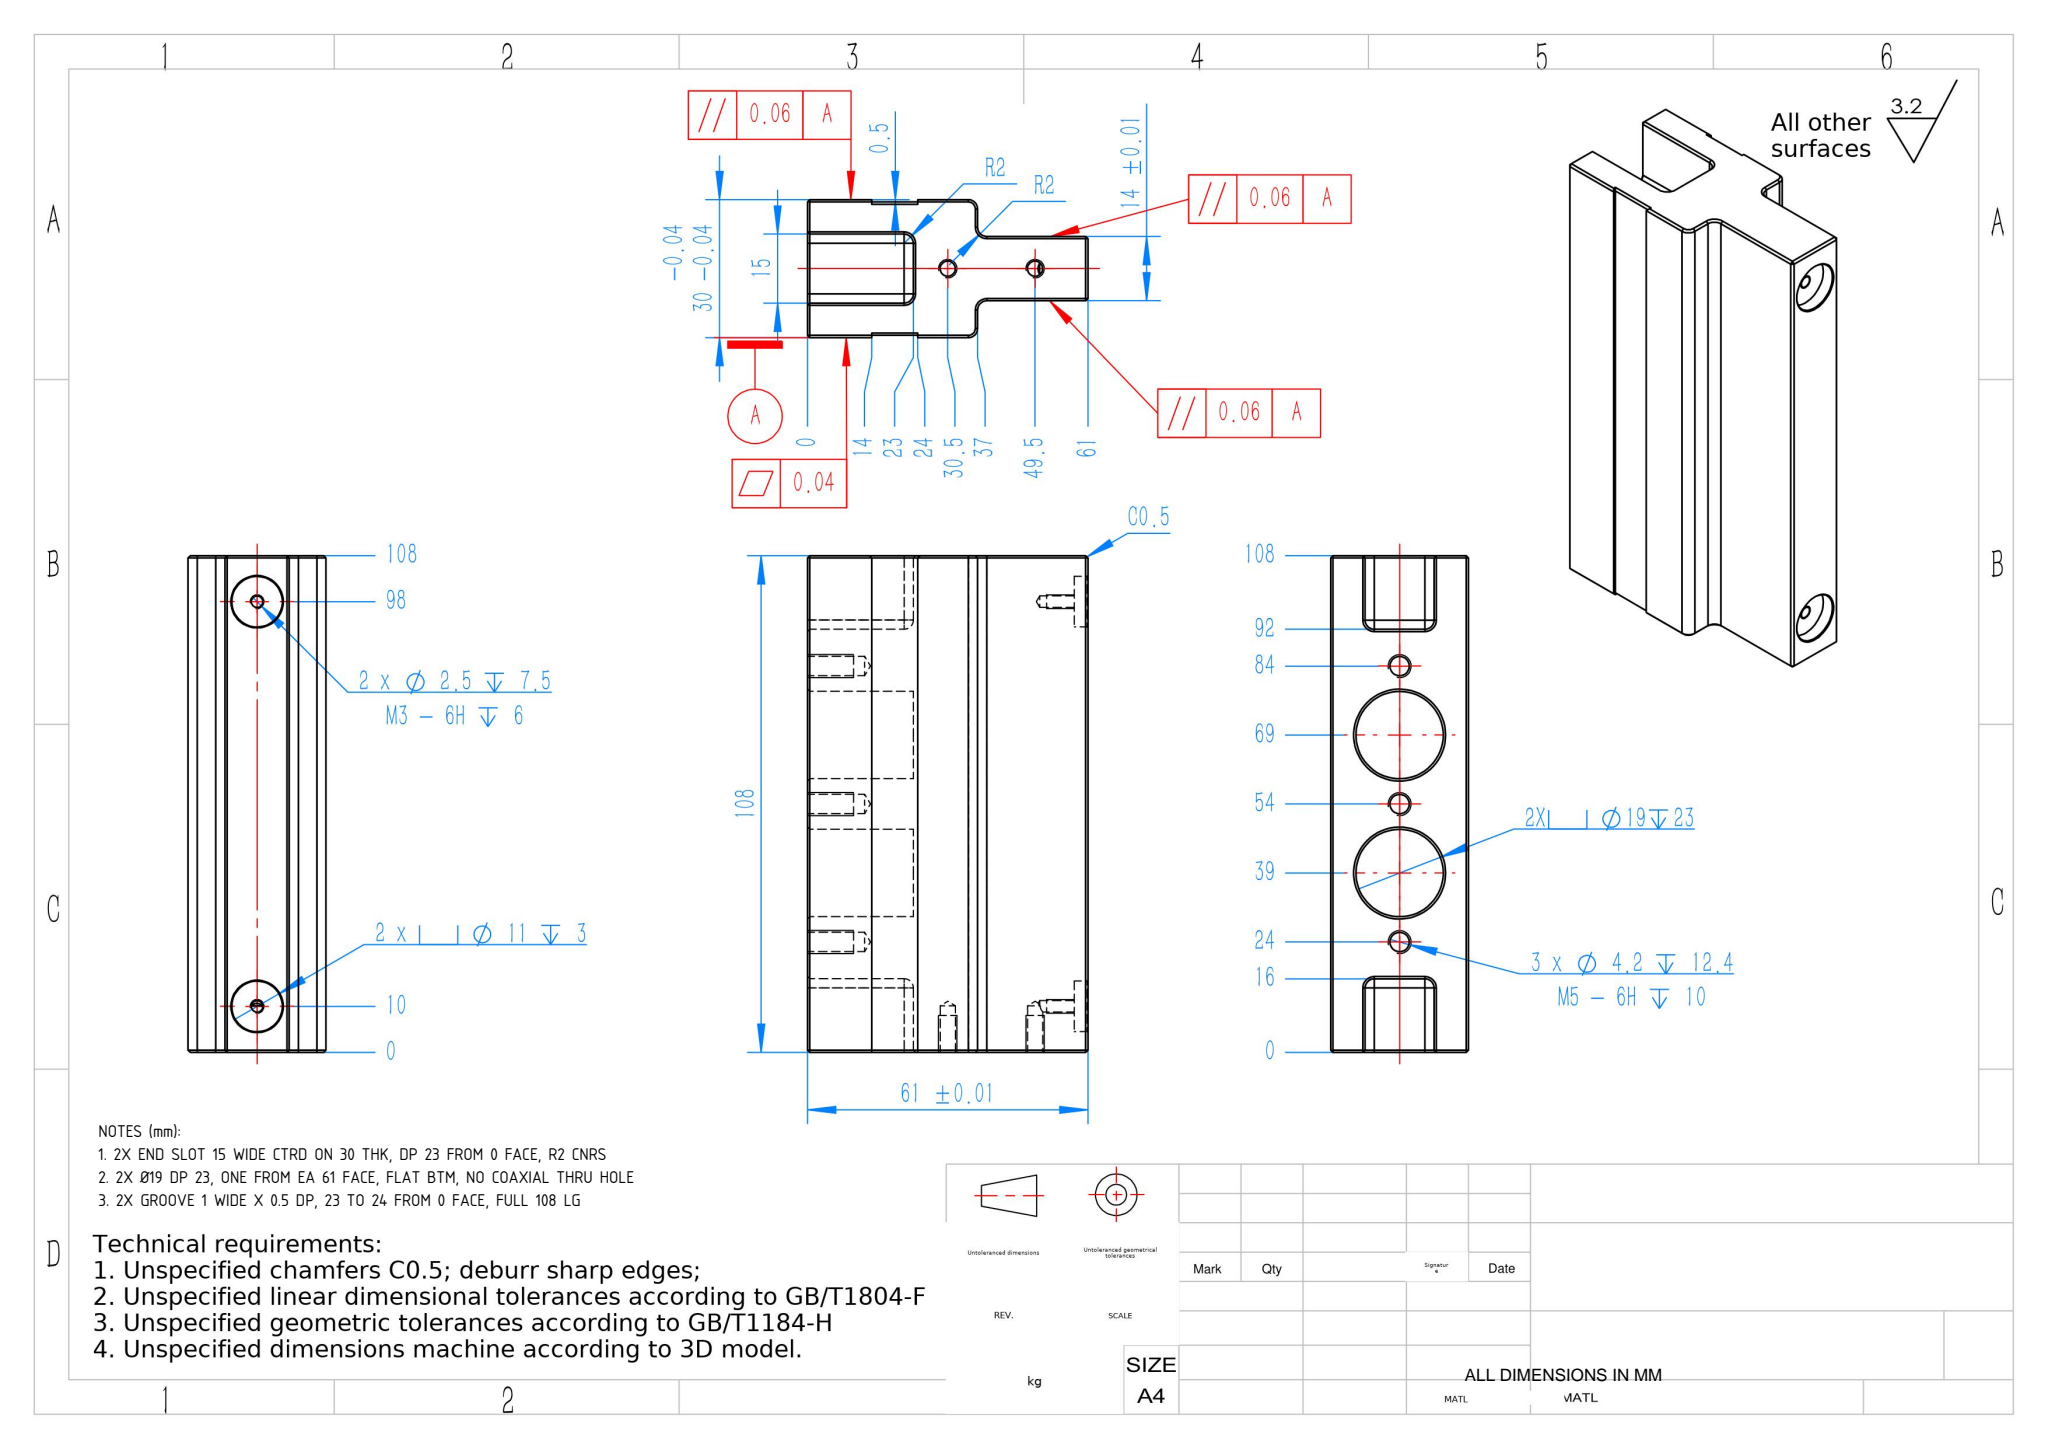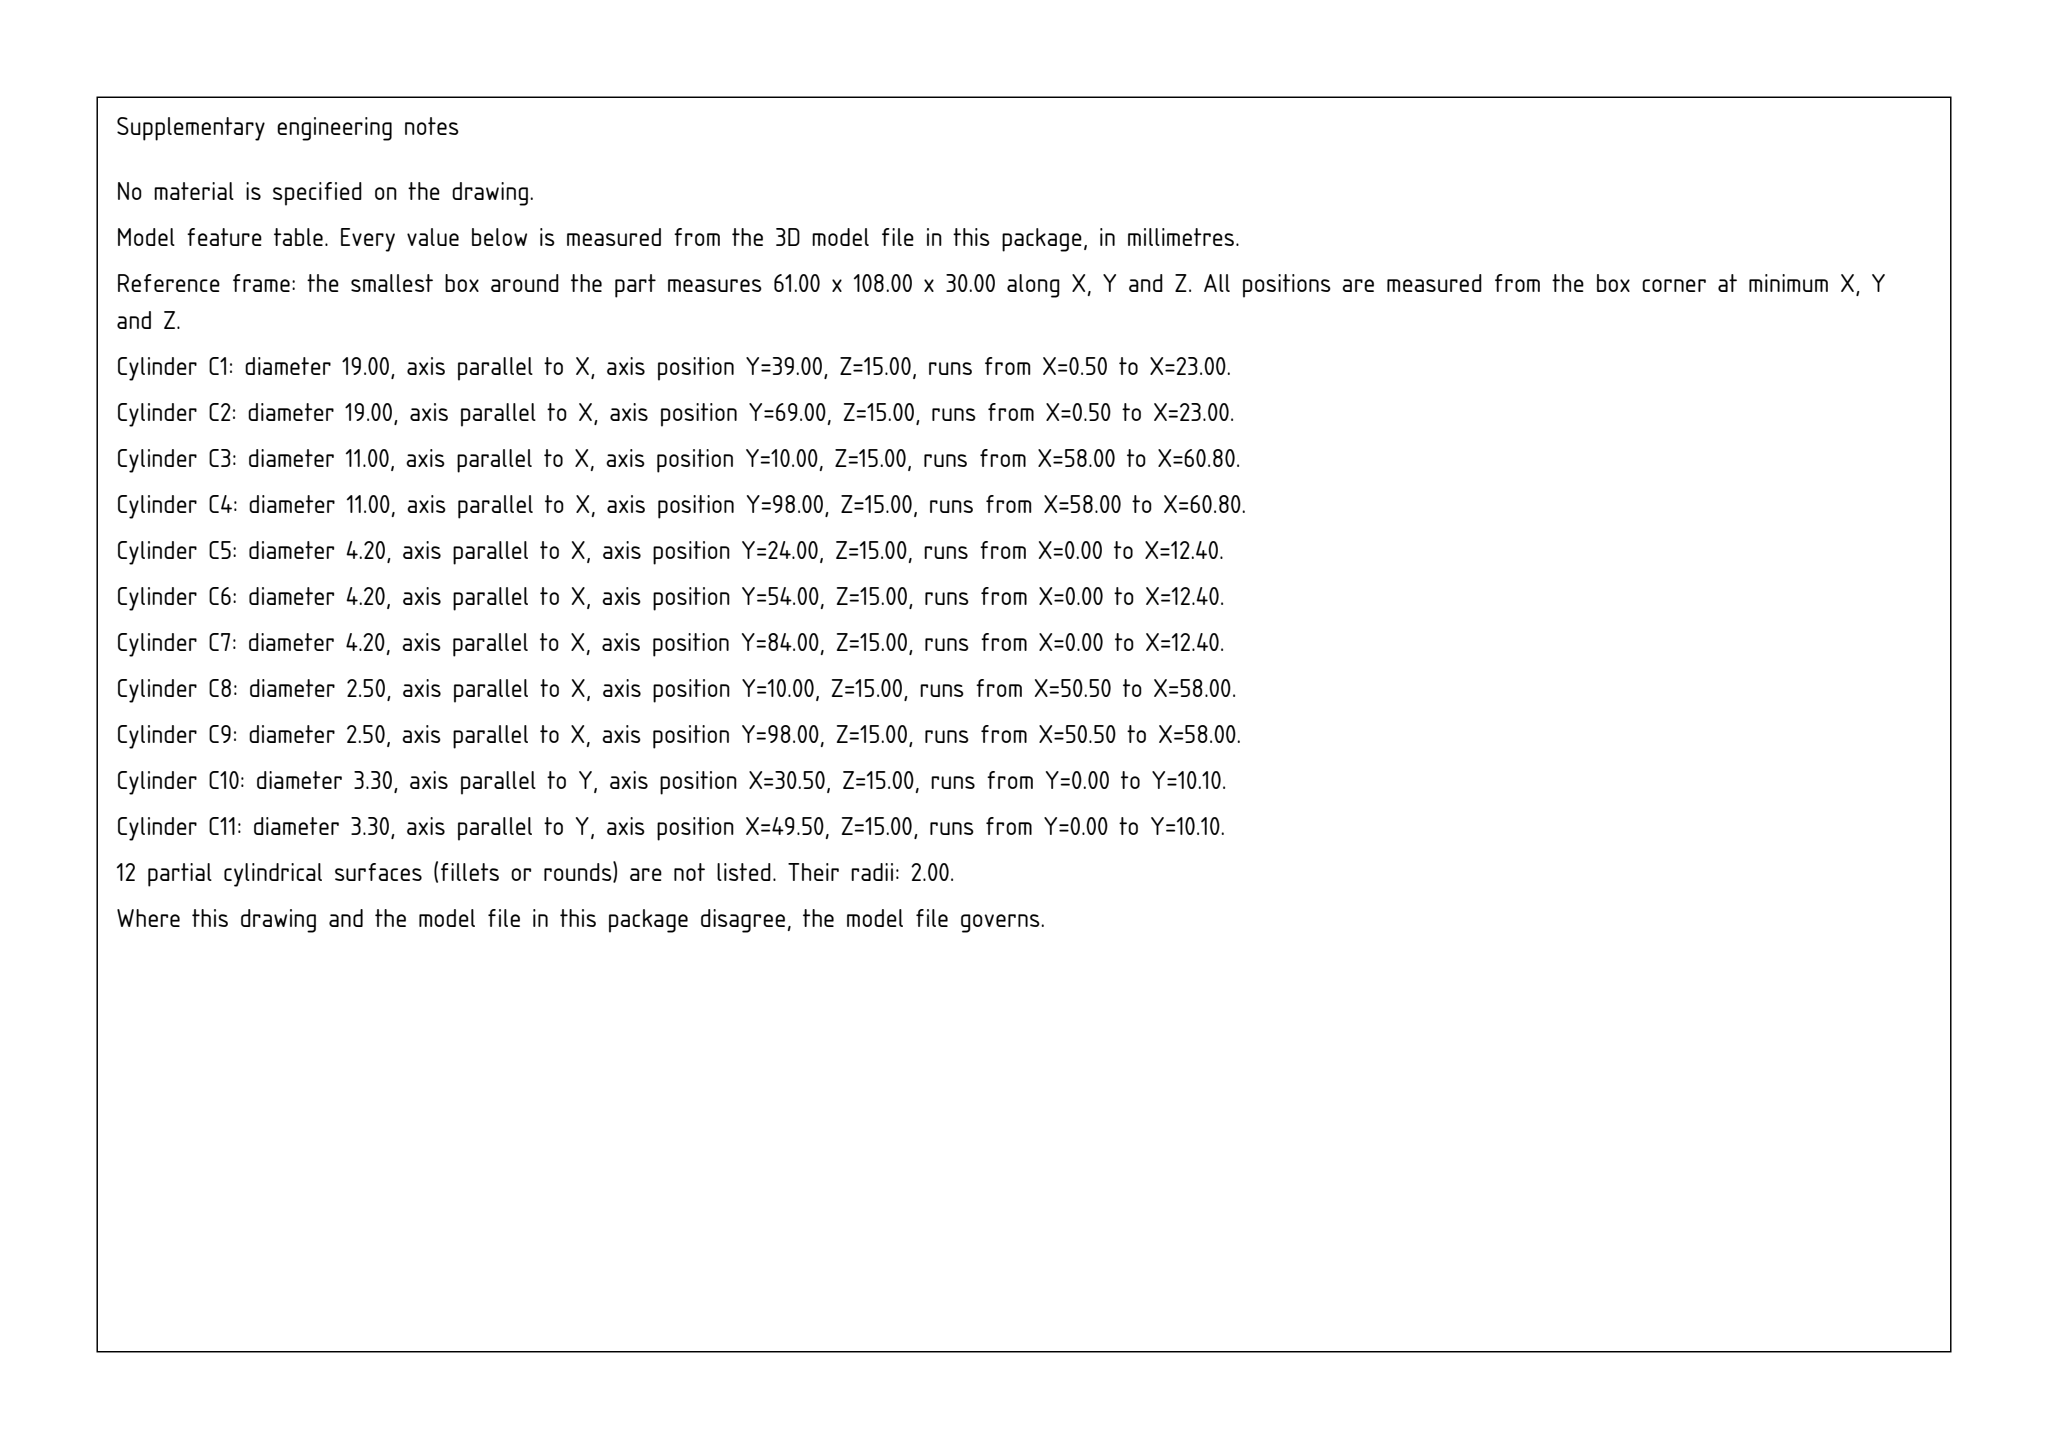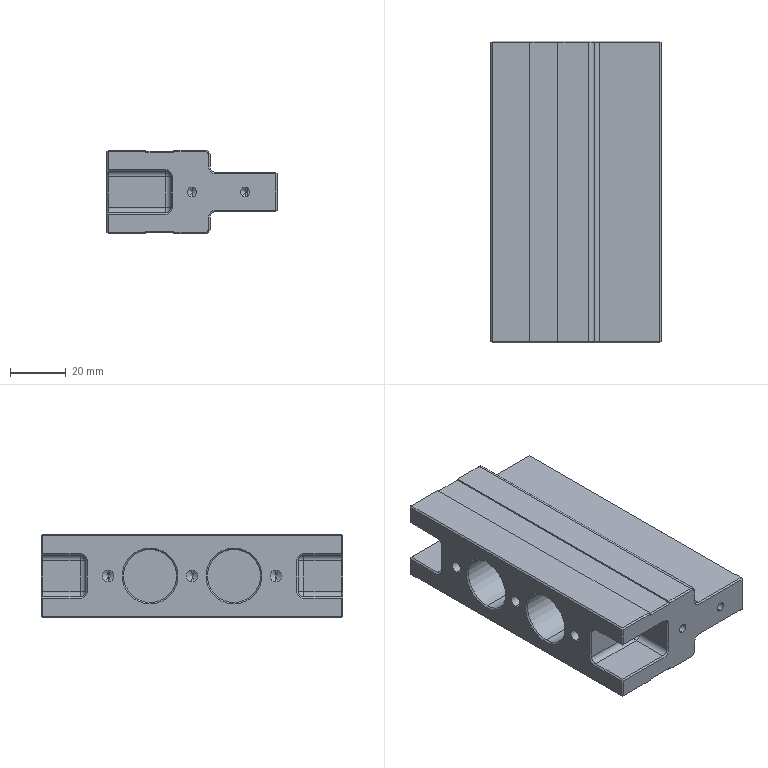Part | SolidWorks | mm | 1 solid | 165 faces | box 61 x 108 x 30 mm | volume 129668 mm3 | plane 88 | cone 37 | cylinder 36 | sphere 4 | commonest cylinder face diameters 4 x14 4.2 x6 19 x4 2.5 x4 11 x4 3.3 x4
Drawing notes:
2X END SLOT 15 WIDE CTRD ON 30 THK, DP 23 FROM 0 FACE, R2 CNRS | from the solid: Pocket walls z=7.5 & 22.5 (15 wide, ctr z=15), floor x=23, ends y=16 & y=92; R2 corner cyls dia4 at (x=21,y=14), (x=21,z=9.5/20.5), (y=14/94,z=9.5/20.5)
2X Ø19 DP 23, ONE FROM EA 61 FACE, FLAT BTM, NO COAXIAL THRU HOLE | from the solid: Ø19 cyls axis x at y=39 & 69, z=15, length 22.5, one per face + 90° chamfer ref dia 19; no smaller coaxial cylinder; 61-2x23=15 solid
2X GROOVE 1 WIDE X 0.5 DP, 23 TO 24 FROM 0 FACE, FULL 108 LG | from the solid: Planes z=0.5 and z=29.5 (0.5 below z=0/30 faces) bounded by planes x=23 and x=24, running full y=0-108